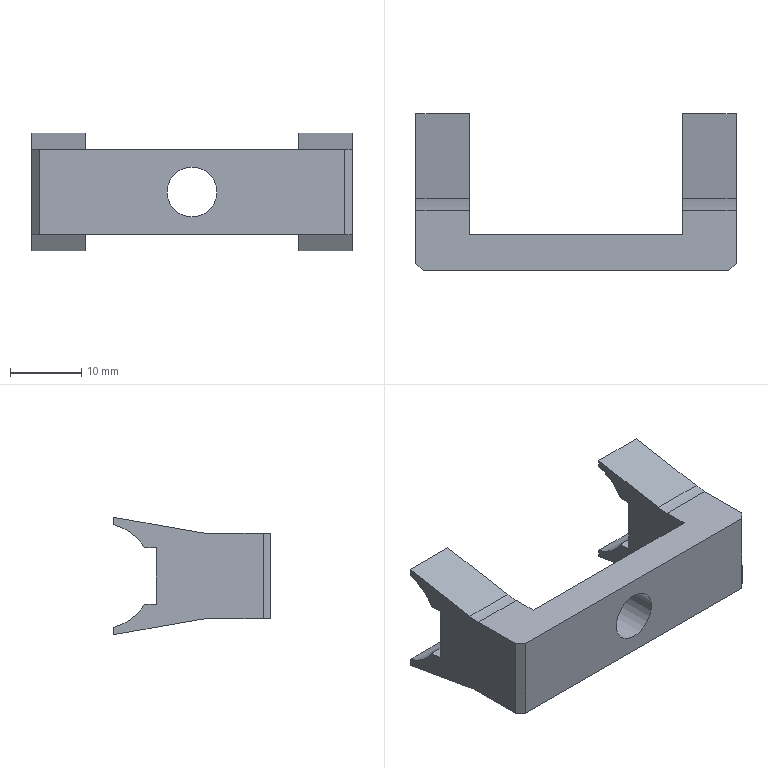Component | SolidWorks | Bracket-1 | 1 solid | 46 faces | box 45 x 22 x 16.5 mm | volume 4506 mm3 | plane 24 | cylinder 14 | cone 8 | commonest cylinder face diameters 5 x4 20 x4 15 x4 7 x2